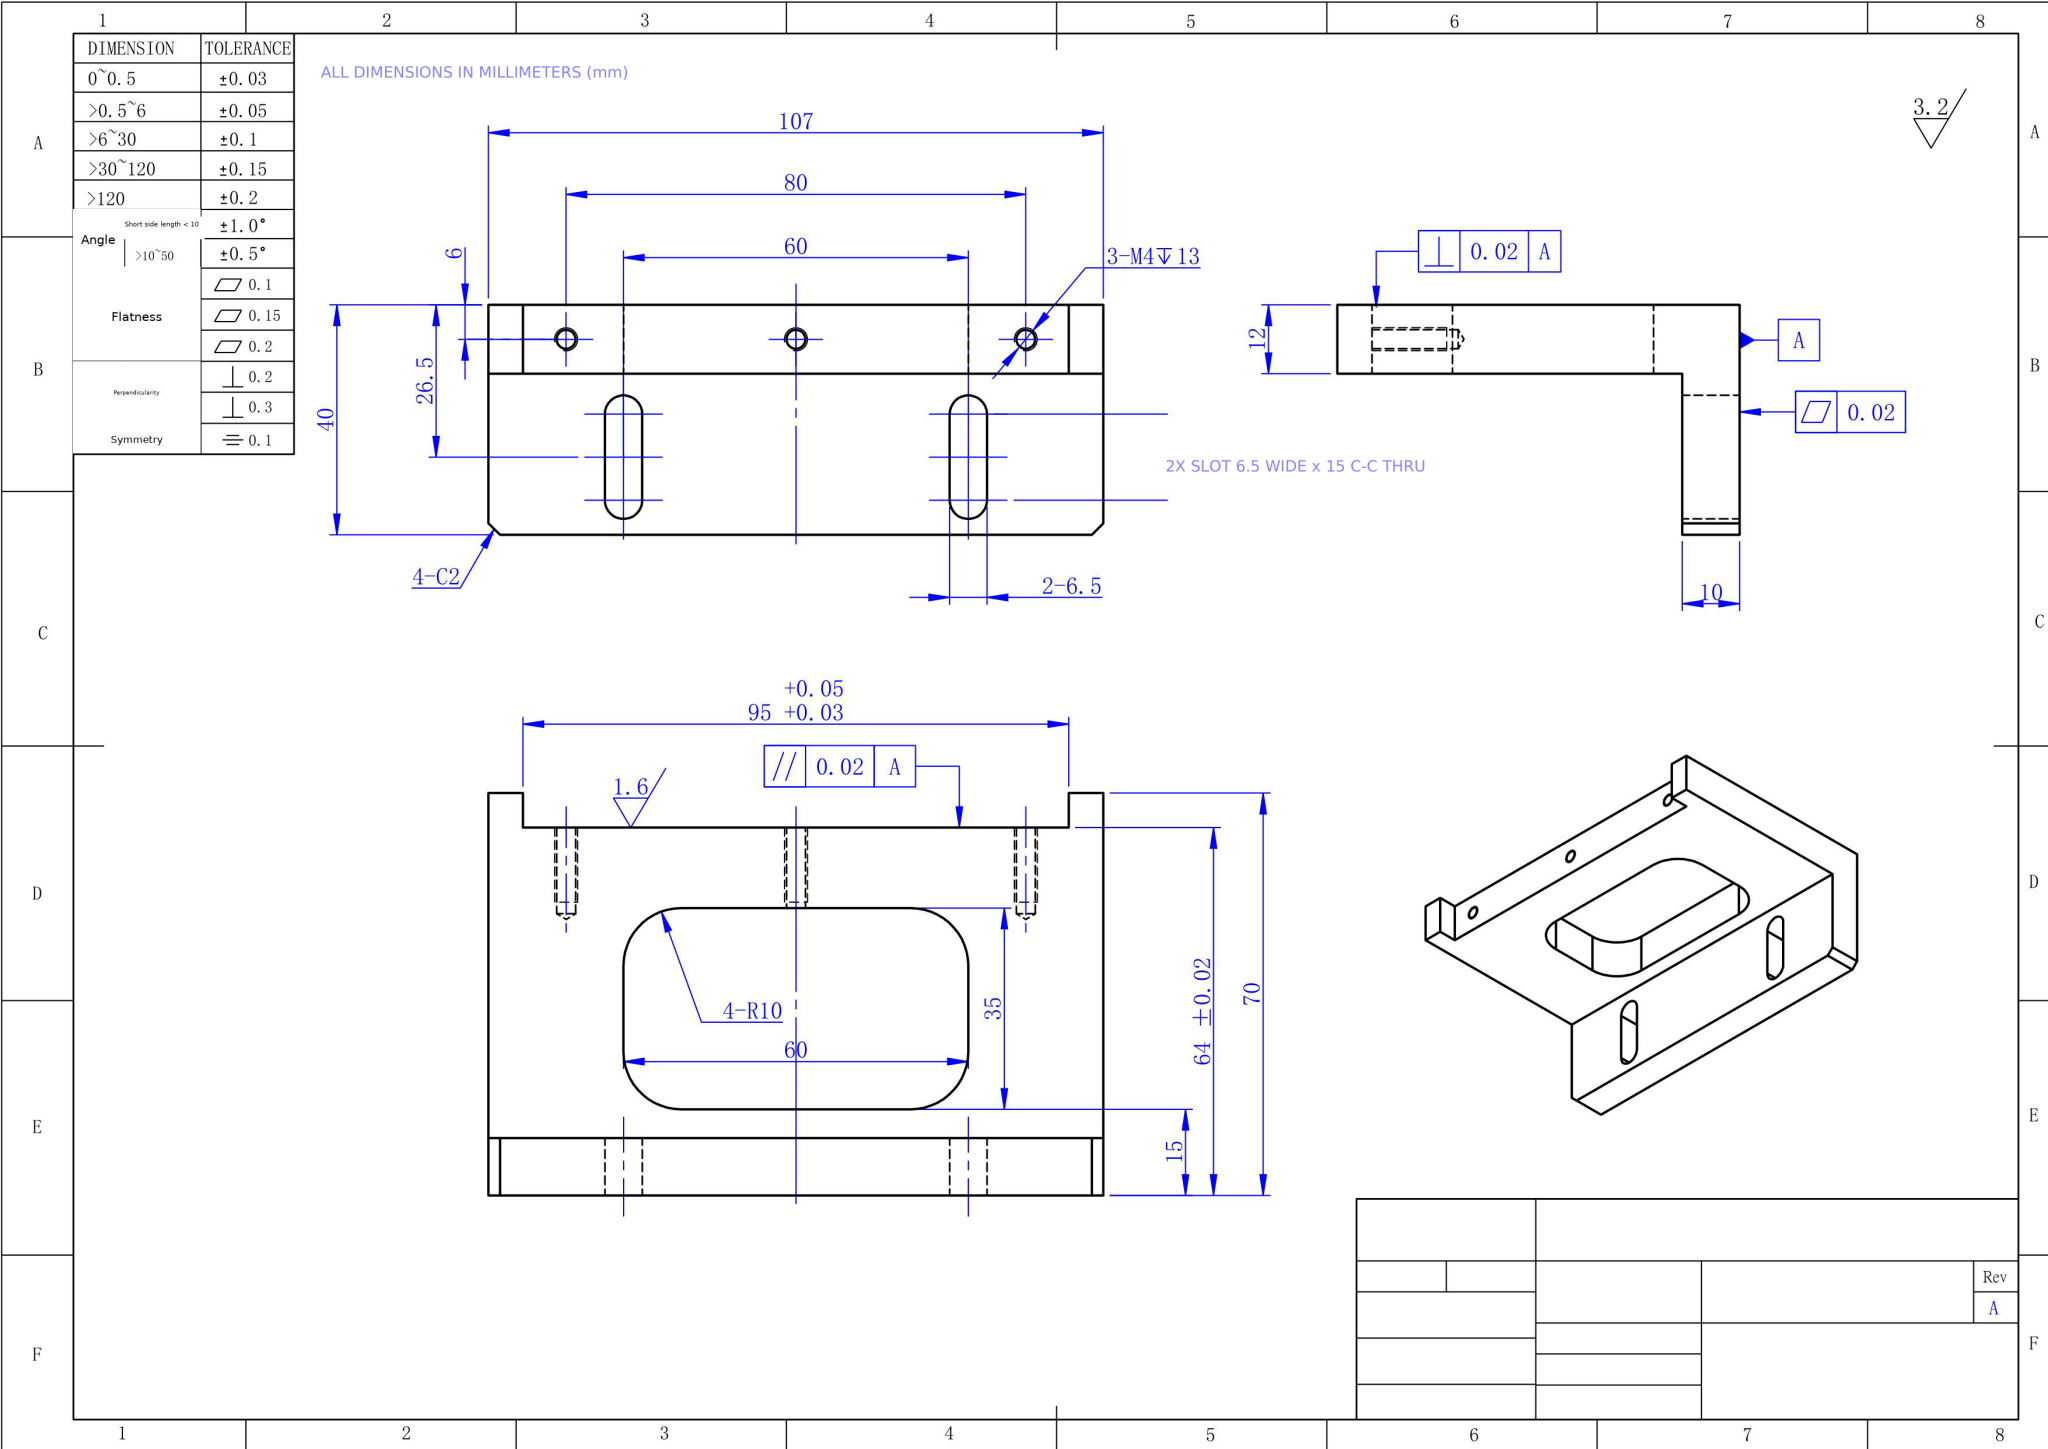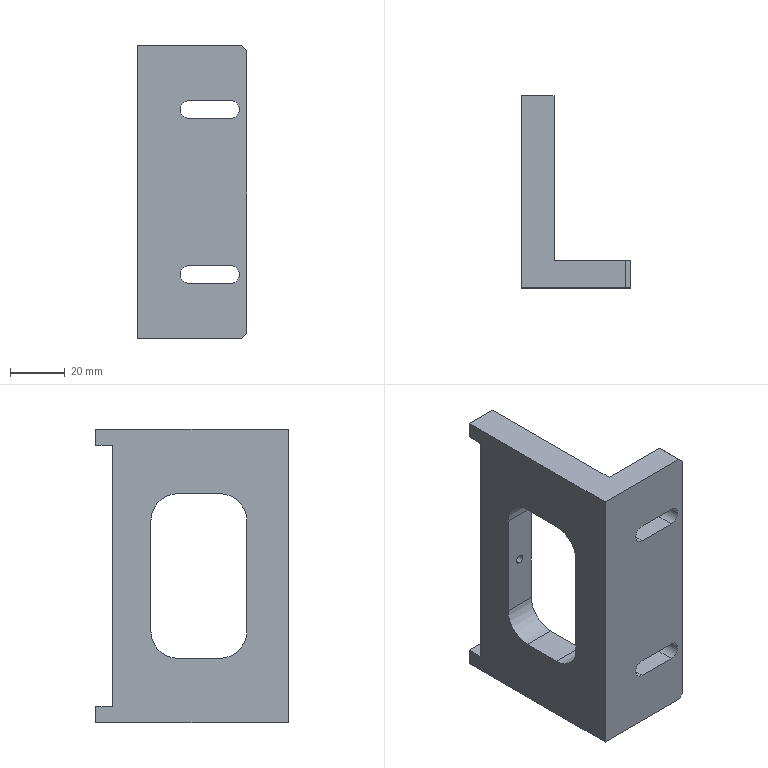Part | NX | mm | 1 solid | 40 faces | box 40 x 70 x 107 mm | volume 85794 mm3 | plane 22 | cylinder 14 | cone 4 | commonest cylinder face diameters 3.3 x6 6.5 x4 20 x4